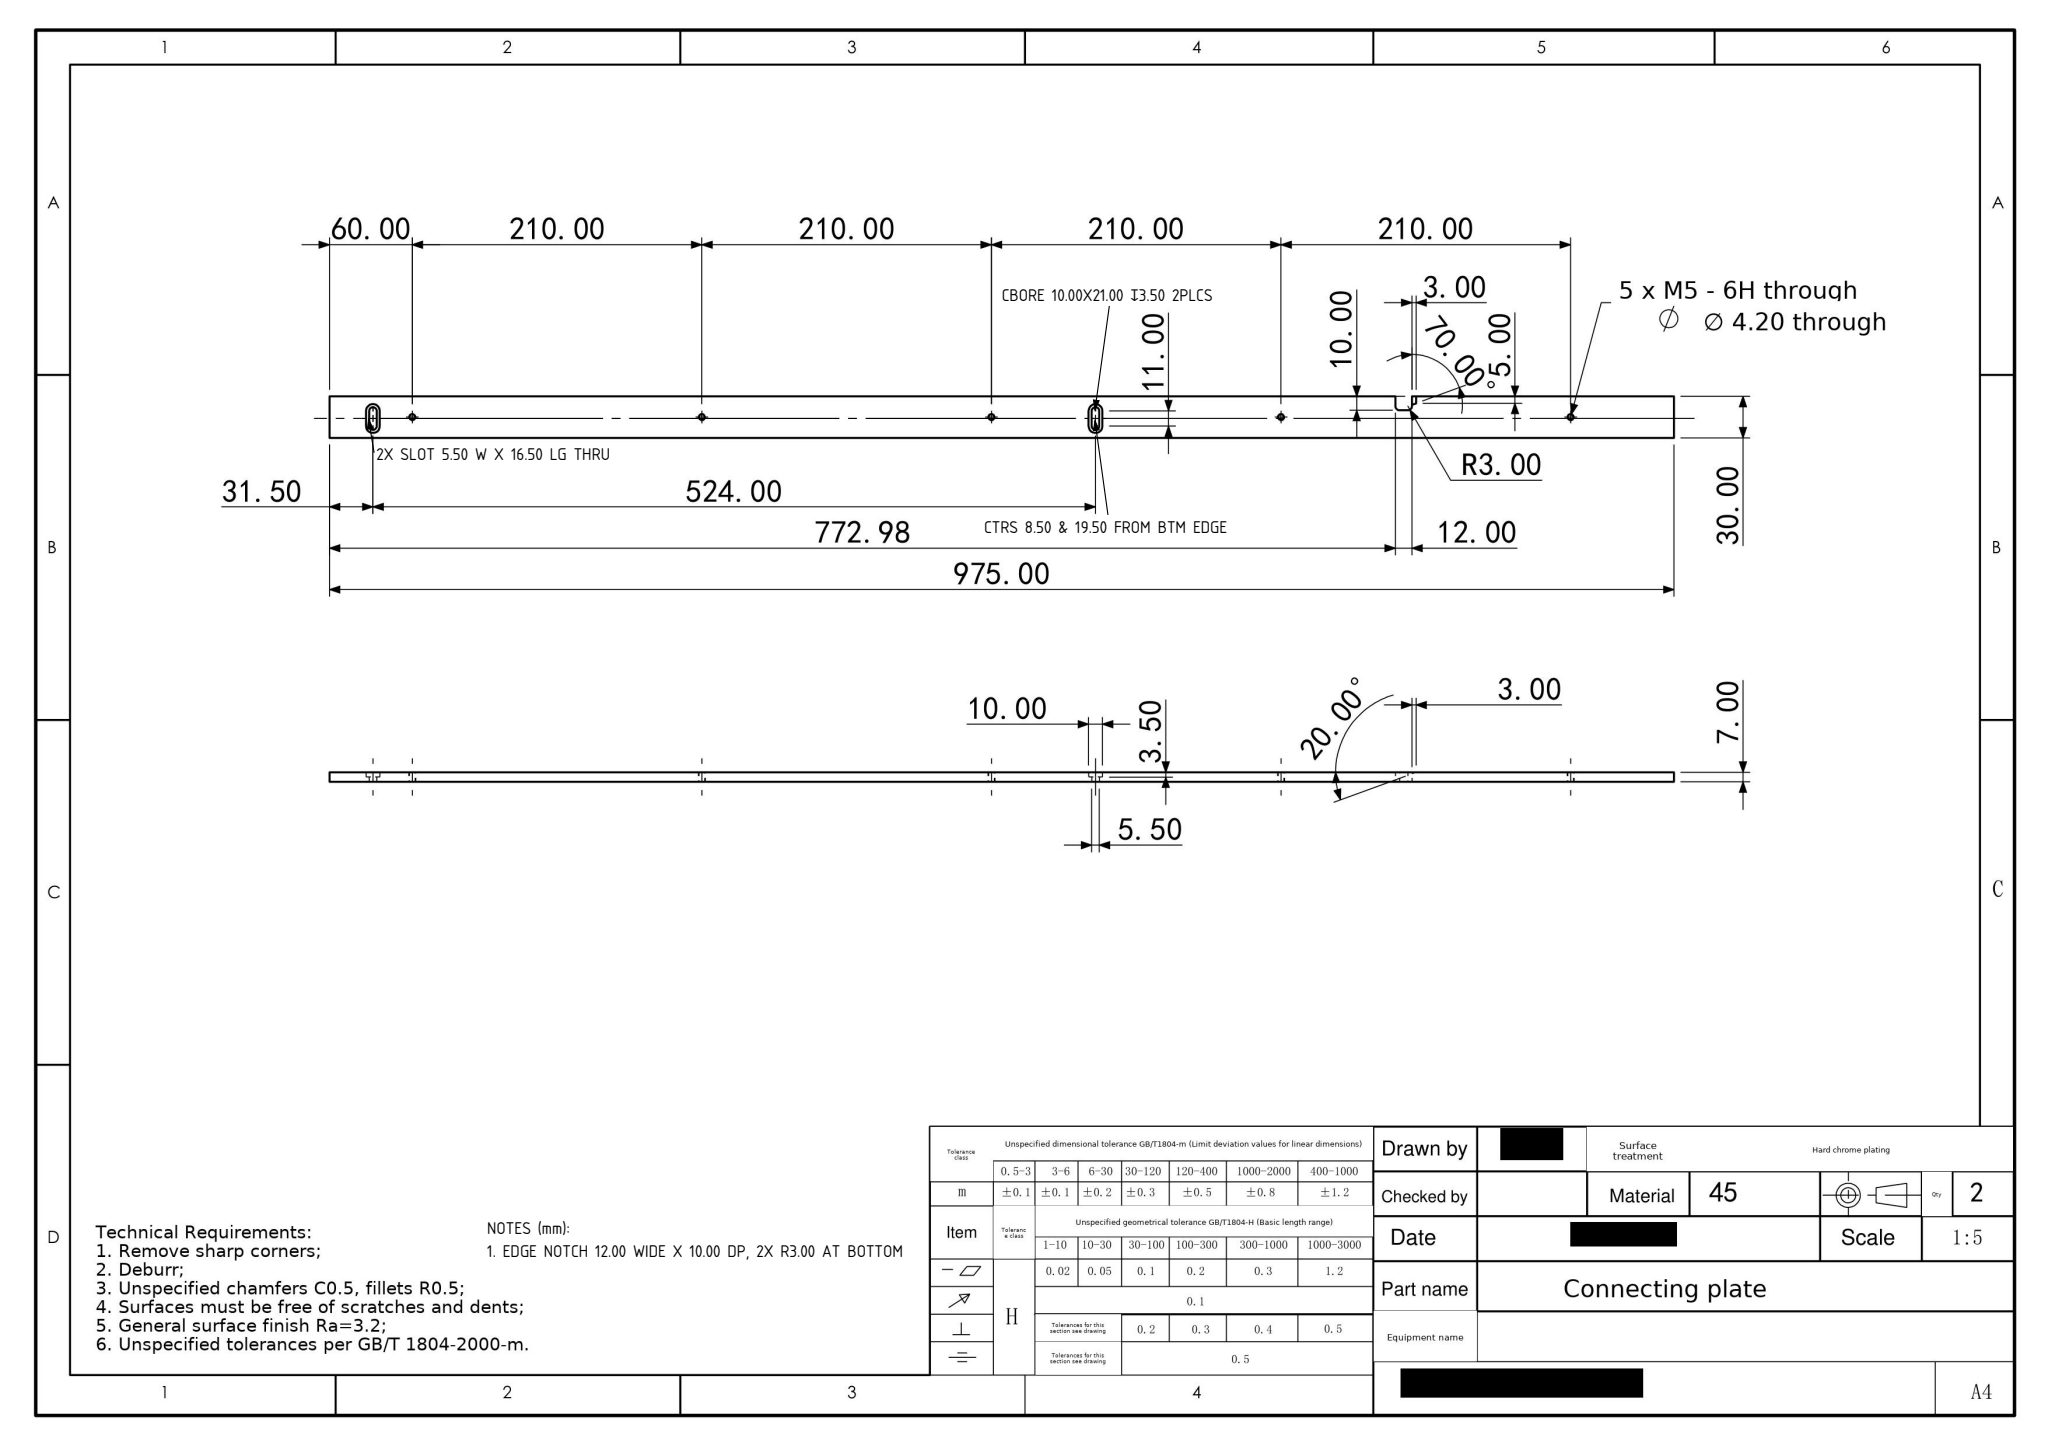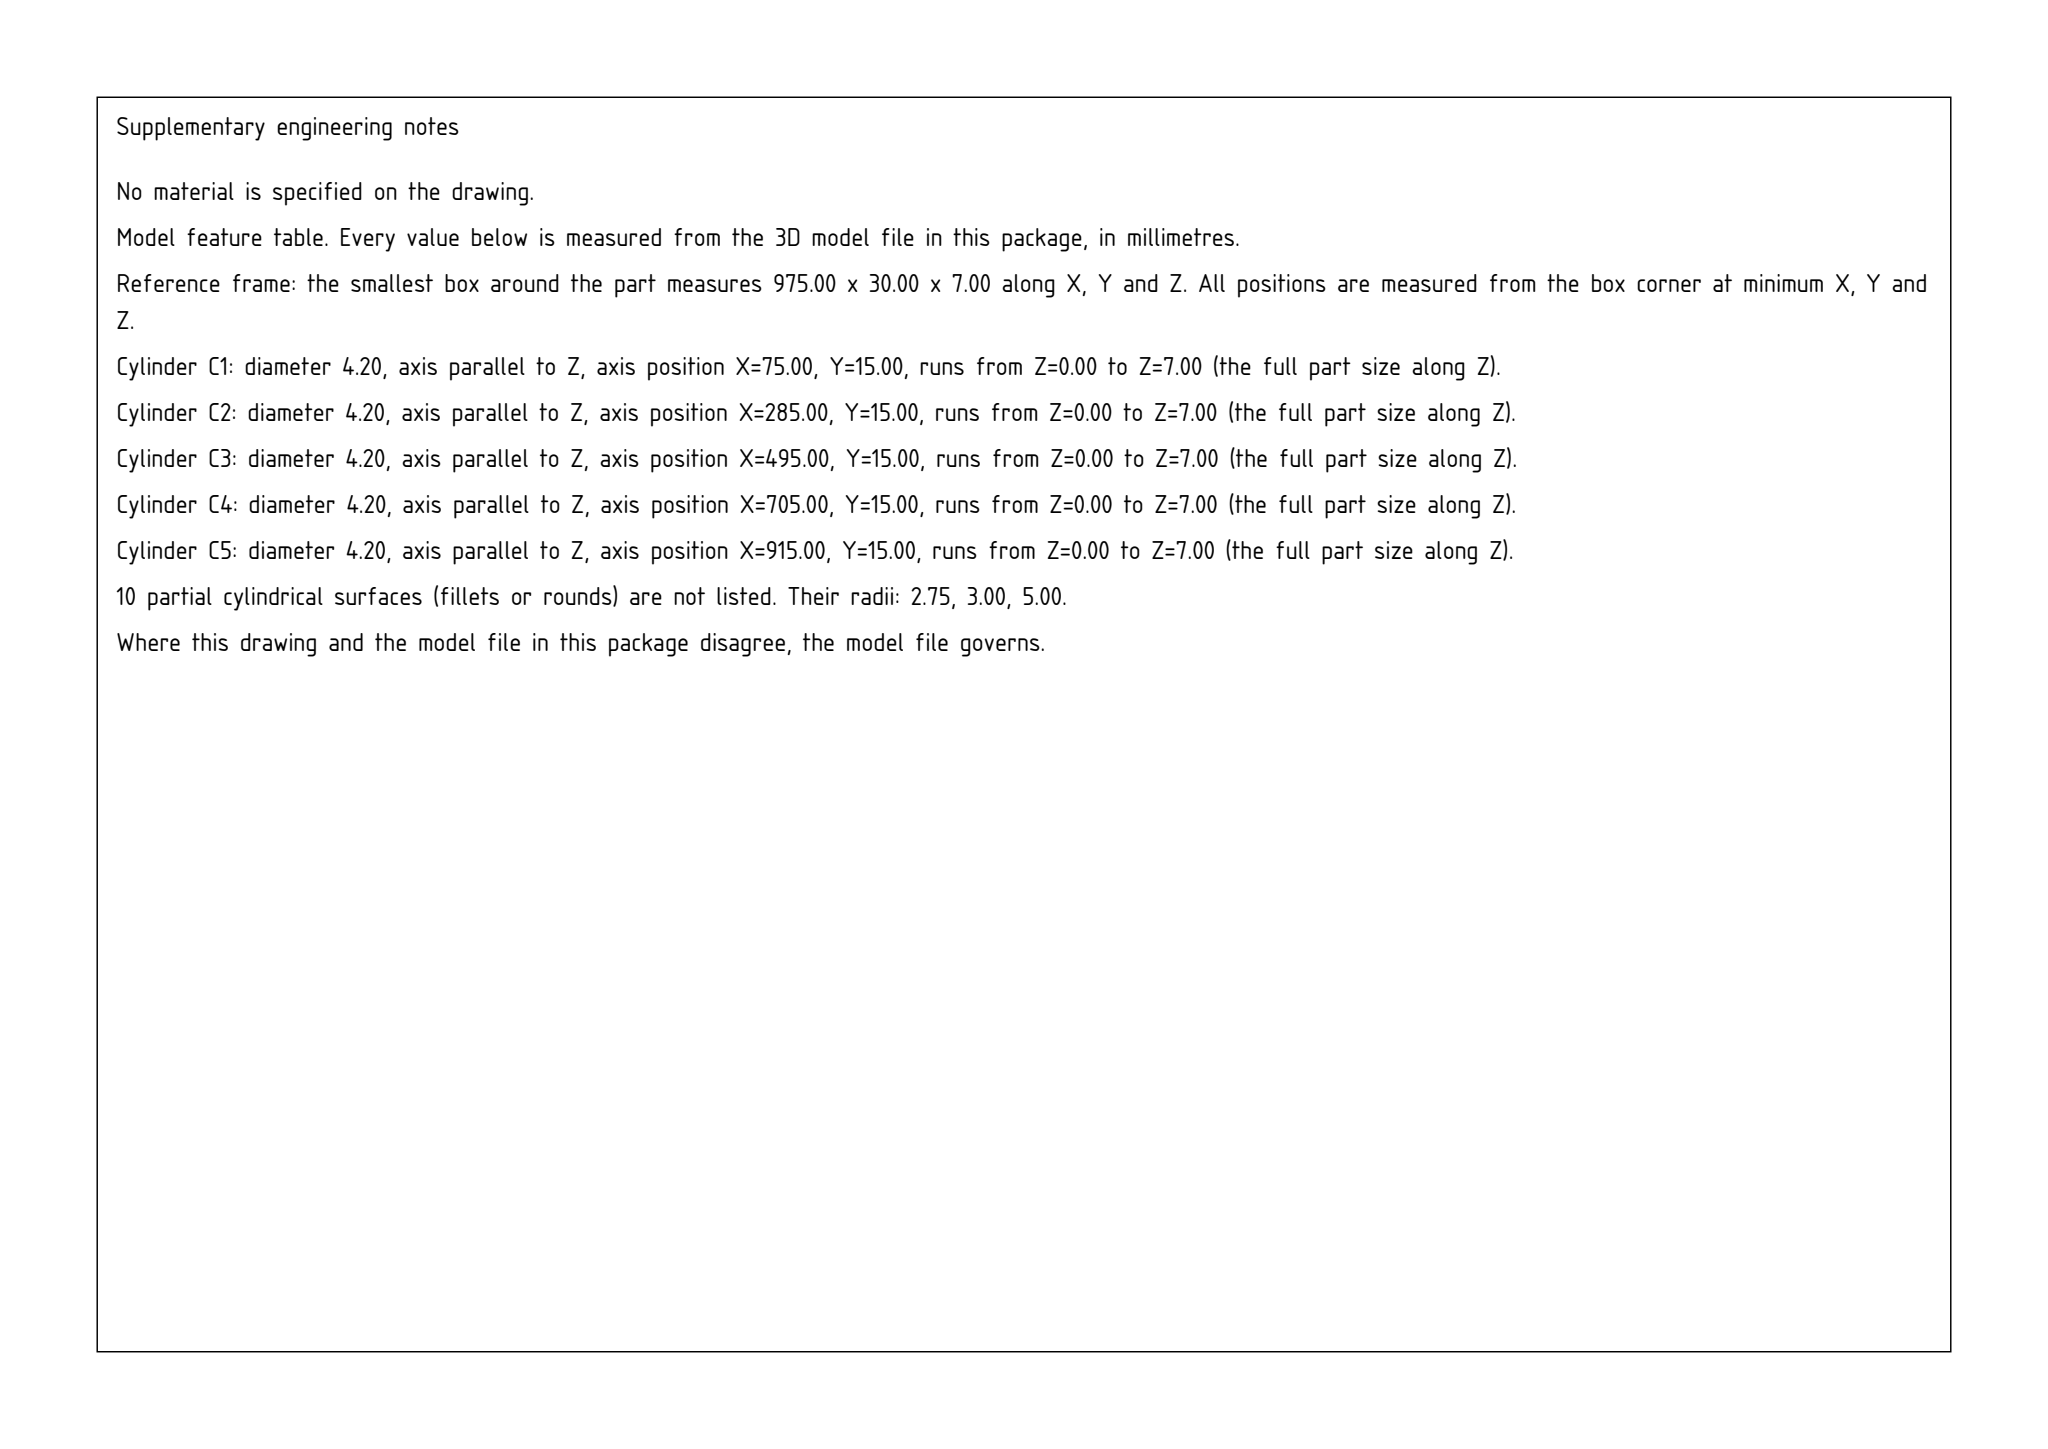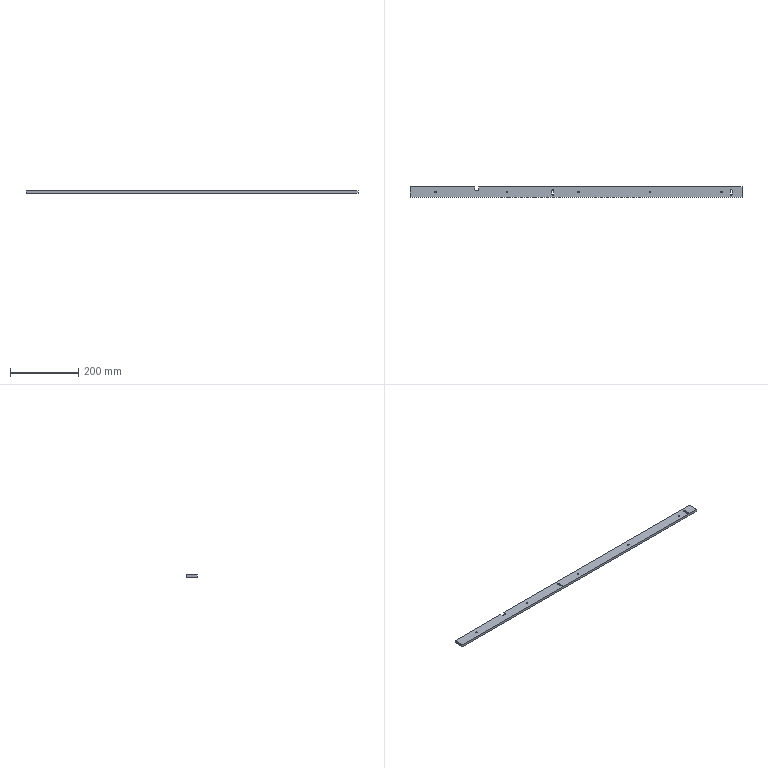Part | SolidWorks | mm | material 45 | 1 solid | 42 faces | box 975 x 30 x 7 mm | volume 201533 mm3 | plane 22 | cylinder 20 | commonest cylinder face diameters 4.2 x10 5.5 x4 10 x4 6 x2
Drawing notes:
2X OBLONG SLOT 5.50 WIDE X 16.50 LG THRU | from the solid: Ø5.5 thru pairs at x=419.5 & 943.5, y=8.5/19.5 (pitch 11) -> 5.5 wide x 16.5 lg
OBLONG CBORE 10.00 WIDE X 21.00 LG X 3.50 DP, 2 PLCS | from the solid: Ø10 cyls at same centers y=8.5/19.5, len 3.5, plane z=3.5 -> 10 x 21 x 3.5 DP
EDGE NOTCH 12.00 WIDE X 10.00 DP, 2X R3.00 AT BOTTOM | from the solid: x planes 190.02 & 202.02 (12 wide), y plane 20.0 vs edge 30.0 (10 DP), 2X Ø6 at y=23.0
2X OBLONG SLOT ARC CTRS 8.50 & 19.50 FROM BOTTOM EDGE (11.00 C-C) | from the solid: Ø5.5/Ø10 slot end cylinders at y=8.5 and y=19.5 (x=419.5 and 943.5); plate y extent 0-30